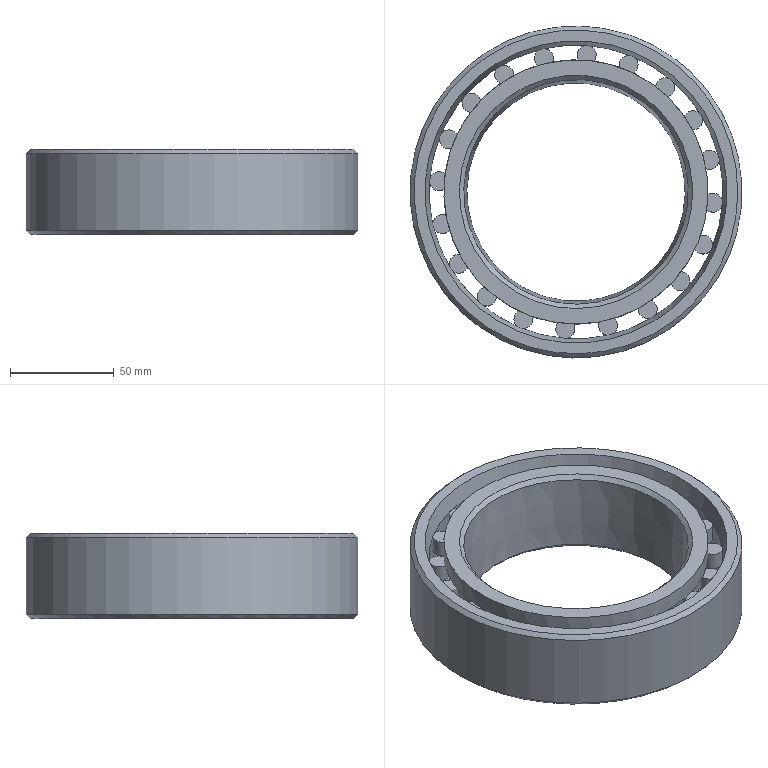Component | NX | CA6140-ZHUZHOU-D3182121 | 42 solids | 142 faces | volume 330939 mm3 | plane 88 | cylinder 47 | cone 7 | commonest cylinder face diameters 9.167 x40 127.333 x3 123.333 x2 160 x1 141.667 x1